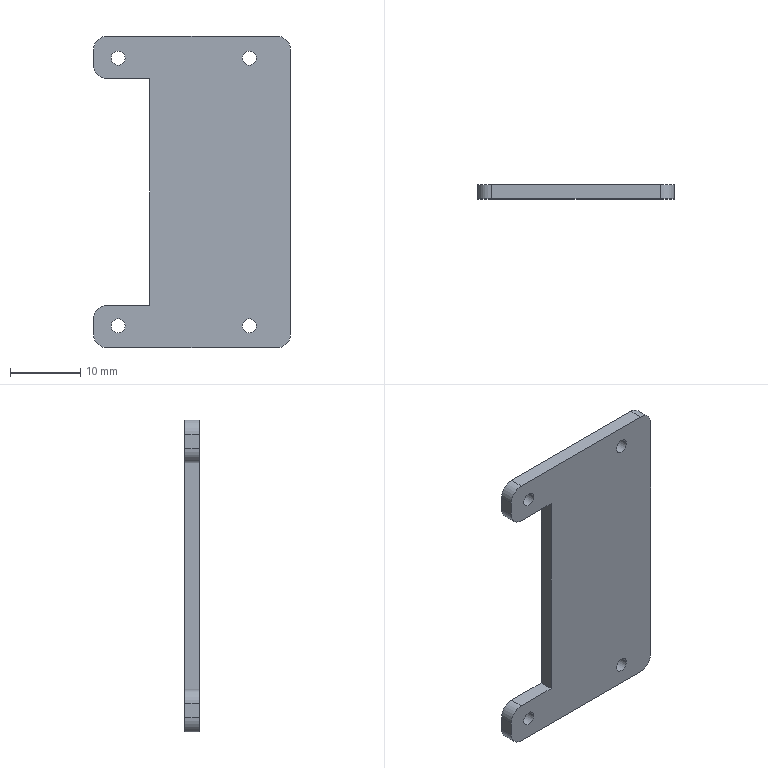Component | SolidWorks | UpperBaffle-1 | 1 solid | 29 faces | box 28.11 x 2 x 44.52 mm | volume 1827 mm3 | plane 15 | cylinder 14 | commonest cylinder face diameters 2 x8 4 x6
build123d program:
from build123d import *

# Parameters (mm, degrees)
BOSS_EXTRUDE1_DEPTH = 2
FILLET1_R           = 2
SKETCH2_R           = 1
CUT_EXTRUDE1_DEPTH  = 10
SKETCH3_W           = 10.322
SKETCH3_H           = 23.58
CUT_EXTRUDE2_DEPTH  = 0.5


with BuildPart() as part:
    # Sketch1 → Boss-Extrude1 (new body)
    with BuildSketch(Plane.XY):
        Polygon((102.385, 21.878), (74.276, 21.878), (74.276, 15.789), (82.305, 15.789), (82.305, -16.558), (74.276, -16.558), (74.276, -22.646), (102.385, -22.646), align=None)
    extrude(amount=BOSS_EXTRUDE1_DEPTH)

    # Fillet1
    fillet1_edges = [part.edges().sort_by_distance(p)[0] for p in [
        (102.385, -22.646, 1),
        (74.276, -22.646, 1),
        (74.276, -16.558, 1),
        (74.276, 15.789, 1),
        (74.276, 21.878, 1),
        (102.385, 21.878, 1),
    ]]
    fillet(fillet1_edges, radius=FILLET1_R)

    # Sketch2 → Cut-Extrude1 (cut)
    with BuildSketch(Plane.XY.offset(2)):
        with Locations((96.517, 18.738)):
            Circle(SKETCH2_R)
        with Locations((77.792, 18.738)):
            Circle(SKETCH2_R)
        with Locations(Location((77.792, -19.506, 0), (0, 0, 180))):
            Circle(SKETCH2_R)
        with Locations(Location((96.517, -19.506, 0), (0, 0, 180))):
            Circle(SKETCH2_R)
    extrude(amount=-CUT_EXTRUDE1_DEPTH, mode=Mode.SUBTRACT)

    # Sketch3 → Cut-Extrude2 (cut)
    with BuildSketch(Plane.XY.offset(2)):
        with Locations((91.241, -0.1111)):
            Rectangle(SKETCH3_W, SKETCH3_H)
    extrude(amount=-CUT_EXTRUDE2_DEPTH, mode=Mode.SUBTRACT)


solid = part.part

# Placed as in the assembly
solid = solid.moved(Location((-18.393, 86.06, 0.5406), (-90, 0, 0)))
STEP:
#1=CARTESIAN_POINT('',(3.115,3.388,0.7893));
#2=VERTEX_POINT('',#1);
#3=CARTESIAN_POINT('',(3.036,3.388,0.7893));
#4=VERTEX_POINT('',#3);
#5=CARTESIAN_POINT('',(3.076,3.388,0.7893));
#6=DIRECTION('',(-0.,-1.,0.));
#7=DIRECTION('',(-1.,0.,0.));
#8=AXIS2_PLACEMENT_3D('',#5,#6,#7);
#9=CIRCLE('',#8,0.03937);
#10=EDGE_CURVE('',#2,#4,#9,.T.);
#11=ORIENTED_EDGE('',*,*,#10,.T.);
#12=CARTESIAN_POINT('',(3.036,3.467,0.7893));
#13=VERTEX_POINT('',#12);
#14=CARTESIAN_POINT('',(3.036,3.073,0.7893));
#15=DIRECTION('',(0.,1.,0.));
#16=VECTOR('',#15,39.37);
#17=LINE('',#14,#16);
#18=EDGE_CURVE('',#4,#13,#17,.T.);
#19=ORIENTED_EDGE('',*,*,#18,.T.);
#20=CARTESIAN_POINT('',(3.115,3.467,0.7893));
#21=VERTEX_POINT('',#20);
#22=CARTESIAN_POINT('',(3.076,3.467,0.7893));
#23=DIRECTION('',(0.,1.,0.));
#24=DIRECTION('',(-1.,0.,0.));
#25=AXIS2_PLACEMENT_3D('',#22,#23,#24);
#26=CIRCLE('',#25,0.03937);
#27=EDGE_CURVE('',#13,#21,#26,.T.);
#28=ORIENTED_EDGE('',*,*,#27,.T.);
#29=CARTESIAN_POINT('',(3.115,3.073,0.7893));
#30=DIRECTION('',(0.,1.,0.));
#31=VECTOR('',#30,39.37);
#32=LINE('',#29,#31);
#33=EDGE_CURVE('',#2,#21,#32,.T.);
#34=ORIENTED_EDGE('',*,*,#33,.F.);
#35=EDGE_LOOP('',(#11,#19,#28,#34));
#36=FACE_OUTER_BOUND('',#35,.T.);
#37=CARTESIAN_POINT('',(3.076,3.073,0.7893));
#38=DIRECTION('',(0.,1.,0.));
#39=DIRECTION('',(1.,0.,0.));
#40=AXIS2_PLACEMENT_3D('',#37,#38,#39);
#41=CYLINDRICAL_SURFACE('',#40,0.03937);
#42=ADVANCED_FACE('',(#36),#41,.F.);
#43=CARTESIAN_POINT('',(2.378,3.388,0.7893));
#44=VERTEX_POINT('',#43);
#45=CARTESIAN_POINT('',(2.299,3.388,0.7893));
#46=VERTEX_POINT('',#45);
#47=CARTESIAN_POINT('',(2.339,3.388,0.7893));
#48=DIRECTION('',(-0.,-1.,0.));
#49=DIRECTION('',(-1.,0.,0.));
#50=AXIS2_PLACEMENT_3D('',#47,#48,#49);
#51=CIRCLE('',#50,0.03937);
#52=EDGE_CURVE('',#44,#46,#51,.T.);
#53=ORIENTED_EDGE('',*,*,#52,.T.);
#54=CARTESIAN_POINT('',(2.299,3.467,0.7893));
#55=VERTEX_POINT('',#54);
#56=CARTESIAN_POINT('',(2.299,3.073,0.7893));
#57=DIRECTION('',(0.,1.,0.));
#58=VECTOR('',#57,39.37);
#59=LINE('',#56,#58);
#60=EDGE_CURVE('',#46,#55,#59,.T.);
#61=ORIENTED_EDGE('',*,*,#60,.T.);
#62=CARTESIAN_POINT('',(2.378,3.467,0.7893));
#63=VERTEX_POINT('',#62);
#64=CARTESIAN_POINT('',(2.339,3.467,0.7893));
#65=DIRECTION('',(0.,1.,0.));
#66=DIRECTION('',(-1.,0.,0.));
#67=AXIS2_PLACEMENT_3D('',#64,#65,#66);
#68=CIRCLE('',#67,0.03937);
#69=EDGE_CURVE('',#55,#63,#68,.T.);
#70=ORIENTED_EDGE('',*,*,#69,.T.);
#71=CARTESIAN_POINT('',(2.378,3.073,0.7893));
#72=DIRECTION('',(0.,1.,0.));
#73=VECTOR('',#72,39.37);
#74=LINE('',#71,#73);
#75=EDGE_CURVE('',#44,#63,#74,.T.);
#76=ORIENTED_EDGE('',*,*,#75,.F.);
#77=EDGE_LOOP('',(#53,#61,#70,#76));
#78=FACE_OUTER_BOUND('',#77,.T.);
#79=CARTESIAN_POINT('',(2.339,3.073,0.7893));
#80=DIRECTION('',(0.,1.,0.));
#81=DIRECTION('',(1.,0.,0.));
#82=AXIS2_PLACEMENT_3D('',#79,#80,#81);
#83=CYLINDRICAL_SURFACE('',#82,0.03937);
#84=ADVANCED_FACE('',(#78),#83,.F.);
#85=CARTESIAN_POINT('',(2.378,3.388,-0.7164));
#86=VERTEX_POINT('',#85);
#87=CARTESIAN_POINT('',(2.299,3.388,-0.7164));
#88=VERTEX_POINT('',#87);
#89=CARTESIAN_POINT('',(2.339,3.388,-0.7164));
#90=DIRECTION('',(-0.,-1.,0.));
#91=DIRECTION('',(-1.,0.,0.));
#92=AXIS2_PLACEMENT_3D('',#89,#90,#91);
#93=CIRCLE('',#92,0.03937);
#94=EDGE_CURVE('',#86,#88,#93,.T.);
#95=ORIENTED_EDGE('',*,*,#94,.T.);
#96=CARTESIAN_POINT('',(2.299,3.467,-0.7164));
#97=VERTEX_POINT('',#96);
#98=CARTESIAN_POINT('',(2.299,3.073,-0.7164));
#99=DIRECTION('',(0.,1.,0.));
#100=VECTOR('',#99,39.37);
#101=LINE('',#98,#100);
#102=EDGE_CURVE('',#88,#97,#101,.T.);
#103=ORIENTED_EDGE('',*,*,#102,.T.);
#104=CARTESIAN_POINT('',(2.378,3.467,-0.7164));
#105=VERTEX_POINT('',#104);
#106=CARTESIAN_POINT('',(2.339,3.467,-0.7164));
#107=DIRECTION('',(0.,1.,0.));
#108=DIRECTION('',(1.,0.,0.));
#109=AXIS2_PLACEMENT_3D('',#106,#107,#108);
#110=CIRCLE('',#109,0.03937);
#111=EDGE_CURVE('',#97,#105,#110,.T.);
#112=ORIENTED_EDGE('',*,*,#111,.T.);
#113=CARTESIAN_POINT('',(2.378,3.073,-0.7164));
#114=DIRECTION('',(0.,1.,0.));
#115=VECTOR('',#114,39.37);
#116=LINE('',#113,#115);
#117=EDGE_CURVE('',#86,#105,#116,.T.);
#118=ORIENTED_EDGE('',*,*,#117,.F.);
#119=EDGE_LOOP('',(#95,#103,#112,#118));
#120=FACE_OUTER_BOUND('',#119,.T.);
#121=CARTESIAN_POINT('',(2.339,3.073,-0.7164));
#122=DIRECTION('',(0.,1.,0.));
#123=DIRECTION('',(1.,0.,0.));
#124=AXIS2_PLACEMENT_3D('',#121,#122,#123);
#125=CYLINDRICAL_SURFACE('',#124,0.03937);
#126=ADVANCED_FACE('',(#120),#125,.F.);
#127=CARTESIAN_POINT('',(3.115,3.388,-0.7164));
#128=VERTEX_POINT('',#127);
#129=CARTESIAN_POINT('',(3.036,3.388,-0.7164));
#130=VERTEX_POINT('',#129);
#131=CARTESIAN_POINT('',(3.076,3.388,-0.7164));
#132=DIRECTION('',(-0.,-1.,0.));
#133=DIRECTION('',(-1.,0.,0.));
#134=AXIS2_PLACEMENT_3D('',#131,#132,#133);
#135=CIRCLE('',#134,0.03937);
#136=EDGE_CURVE('',#128,#130,#135,.T.);
#137=ORIENTED_EDGE('',*,*,#136,.T.);
#138=CARTESIAN_POINT('',(3.036,3.467,-0.7164));
#139=VERTEX_POINT('',#138);
#140=CARTESIAN_POINT('',(3.036,3.073,-0.7164));
#141=DIRECTION('',(0.,1.,0.));
#142=VECTOR('',#141,39.37);
#143=LINE('',#140,#142);
#144=EDGE_CURVE('',#130,#139,#143,.T.);
#145=ORIENTED_EDGE('',*,*,#144,.T.);
#146=CARTESIAN_POINT('',(3.115,3.467,-0.7164));
#147=VERTEX_POINT('',#146);
#148=CARTESIAN_POINT('',(3.076,3.467,-0.7164));
#149=DIRECTION('',(0.,1.,0.));
#150=DIRECTION('',(1.,0.,0.));
#151=AXIS2_PLACEMENT_3D('',#148,#149,#150);
#152=CIRCLE('',#151,0.03937);
#153=EDGE_CURVE('',#139,#147,#152,.T.);
#154=ORIENTED_EDGE('',*,*,#153,.T.);
#155=CARTESIAN_POINT('',(3.115,3.073,-0.7164));
#156=DIRECTION('',(0.,1.,0.));
#157=VECTOR('',#156,39.37);
#158=LINE('',#155,#157);
#159=EDGE_CURVE('',#128,#147,#158,.T.);
#160=ORIENTED_EDGE('',*,*,#159,.F.);
#161=EDGE_LOOP('',(#137,#145,#154,#160));
#162=FACE_OUTER_BOUND('',#161,.T.);
#163=CARTESIAN_POINT('',(3.076,3.073,-0.7164));
#164=DIRECTION('',(0.,1.,0.));
#165=DIRECTION('',(1.,0.,0.));
#166=AXIS2_PLACEMENT_3D('',#163,#164,#165);
#167=CYLINDRICAL_SURFACE('',#166,0.03937);
#168=ADVANCED_FACE('',(#162),#167,.F.);
#169=CARTESIAN_POINT('',(3.307,3.467,0.8341));
#170=VERTEX_POINT('',#169);
#171=CARTESIAN_POINT('',(3.307,3.467,-0.7613));
#172=VERTEX_POINT('',#171);
#173=CARTESIAN_POINT('',(3.307,3.467,-0.84));
#174=DIRECTION('',(0.,0.,-1.));
#175=VECTOR('',#174,39.37);
#176=LINE('',#173,#175);
#177=EDGE_CURVE('',#170,#172,#176,.T.);
#178=ORIENTED_EDGE('',*,*,#177,.F.);
#179=CARTESIAN_POINT('',(3.307,3.388,0.8341));
#180=VERTEX_POINT('',#179);
#181=CARTESIAN_POINT('',(3.307,3.467,0.8341));
#182=DIRECTION('',(-0.,-1.,0.));
#183=VECTOR('',#182,39.37);
#184=LINE('',#181,#183);
#185=EDGE_CURVE('',#170,#180,#184,.T.);
#186=ORIENTED_EDGE('',*,*,#185,.T.);
#187=CARTESIAN_POINT('',(3.307,3.388,-0.7613));
#188=VERTEX_POINT('',#187);
#189=CARTESIAN_POINT('',(3.307,3.388,-0.84));
#190=DIRECTION('',(0.,0.,-1.));
#191=VECTOR('',#190,39.37);
#192=LINE('',#189,#191);
#193=EDGE_CURVE('',#180,#188,#192,.T.);
#194=ORIENTED_EDGE('',*,*,#193,.T.);
#195=CARTESIAN_POINT('',(3.307,3.467,-0.7613));
#196=DIRECTION('',(0.,1.,0.));
#197=VECTOR('',#196,39.37);
#198=LINE('',#195,#197);
#199=EDGE_CURVE('',#188,#172,#198,.T.);
#200=ORIENTED_EDGE('',*,*,#199,.T.);
#201=EDGE_LOOP('',(#178,#186,#194,#200));
#202=FACE_OUTER_BOUND('',#201,.T.);
#203=CARTESIAN_POINT('',(3.307,3.467,-0.84));
#204=DIRECTION('',(-1.,0.,0.));
#205=DIRECTION('',(0.,1.,0.));
#206=AXIS2_PLACEMENT_3D('',#203,#204,#205);
#207=PLANE('',#206);
#208=ADVANCED_FACE('',(#202),#207,.F.);
#209=CARTESIAN_POINT('',(3.228,3.388,-0.84));
#210=VERTEX_POINT('',#209);
#211=CARTESIAN_POINT('',(2.279,3.388,-0.84));
#212=VERTEX_POINT('',#211);
#213=CARTESIAN_POINT('',(3.307,3.388,-0.84));
#214=DIRECTION('',(-1.,0.,-0.));
#215=VECTOR('',#214,39.37);
#216=LINE('',#213,#215);
#217=EDGE_CURVE('',#210,#212,#216,.T.);
#218=ORIENTED_EDGE('',*,*,#217,.T.);
#219=CARTESIAN_POINT('',(2.279,3.467,-0.84));
#220=VERTEX_POINT('',#219);
#221=CARTESIAN_POINT('',(2.279,3.467,-0.84));
#222=DIRECTION('',(0.,1.,0.));
#223=VECTOR('',#222,39.37);
#224=LINE('',#221,#223);
#225=EDGE_CURVE('',#212,#220,#224,.T.);
#226=ORIENTED_EDGE('',*,*,#225,.T.);
#227=CARTESIAN_POINT('',(3.228,3.467,-0.84));
#228=VERTEX_POINT('',#227);
#229=CARTESIAN_POINT('',(3.307,3.467,-0.84));
#230=DIRECTION('',(-1.,0.,-0.));
#231=VECTOR('',#230,39.37);
#232=LINE('',#229,#231);
#233=EDGE_CURVE('',#228,#220,#232,.T.);
#234=ORIENTED_EDGE('',*,*,#233,.F.);
#235=CARTESIAN_POINT('',(3.228,3.467,-0.84));
#236=DIRECTION('',(-0.,-1.,0.));
#237=VECTOR('',#236,39.37);
#238=LINE('',#235,#237);
#239=EDGE_CURVE('',#228,#210,#238,.T.);
#240=ORIENTED_EDGE('',*,*,#239,.T.);
#241=EDGE_LOOP('',(#218,#226,#234,#240));
#242=FACE_OUTER_BOUND('',#241,.T.);
#243=CARTESIAN_POINT('',(3.307,3.467,-0.84));
#244=DIRECTION('',(-0.,0.,1.));
#245=DIRECTION('',(1.,-0.,0.));
#246=AXIS2_PLACEMENT_3D('',#243,#244,#245);
#247=PLANE('',#246);
#248=ADVANCED_FACE('',(#242),#247,.F.);
#249=CARTESIAN_POINT('',(2.2,3.388,-0.7613));
#250=VERTEX_POINT('',#249);
#251=CARTESIAN_POINT('',(2.2,3.388,-0.6791));
#252=VERTEX_POINT('',#251);
#253=CARTESIAN_POINT('',(2.2,3.388,-0.84));
#254=DIRECTION('',(0.,0.,1.));
#255=VECTOR('',#254,39.37);
#256=LINE('',#253,#255);
#257=EDGE_CURVE('',#250,#252,#256,.T.);
#258=ORIENTED_EDGE('',*,*,#257,.T.);
#259=CARTESIAN_POINT('',(2.2,3.467,-0.6791));
#260=VERTEX_POINT('',#259);
#261=CARTESIAN_POINT('',(2.2,3.467,-0.6791));
#262=DIRECTION('',(0.,1.,0.));
#263=VECTOR('',#262,39.37);
#264=LINE('',#261,#263);
#265=EDGE_CURVE('',#252,#260,#264,.T.);
#266=ORIENTED_EDGE('',*,*,#265,.T.);
#267=CARTESIAN_POINT('',(2.2,3.467,-0.7613));
#268=VERTEX_POINT('',#267);
#269=CARTESIAN_POINT('',(2.2,3.467,-0.84));
#270=DIRECTION('',(0.,0.,1.));
#271=VECTOR('',#270,39.37);
#272=LINE('',#269,#271);
#273=EDGE_CURVE('',#268,#260,#272,.T.);
#274=ORIENTED_EDGE('',*,*,#273,.F.);
#275=CARTESIAN_POINT('',(2.2,3.467,-0.7613));
#276=DIRECTION('',(-0.,-1.,0.));
#277=VECTOR('',#276,39.37);
#278=LINE('',#275,#277);
#279=EDGE_CURVE('',#268,#250,#278,.T.);
#280=ORIENTED_EDGE('',*,*,#279,.T.);
#281=EDGE_LOOP('',(#258,#266,#274,#280));
#282=FACE_OUTER_BOUND('',#281,.T.);
#283=CARTESIAN_POINT('',(2.2,3.467,-0.84));
#284=DIRECTION('',(1.,-0.,0.));
#285=DIRECTION('',(-0.,-1.,0.));
#286=AXIS2_PLACEMENT_3D('',#283,#284,#285);
#287=PLANE('',#286);
#288=ADVANCED_FACE('',(#282),#287,.F.);
#289=CARTESIAN_POINT('',(2.279,3.467,-0.6003));
#290=VERTEX_POINT('',#289);
#291=CARTESIAN_POINT('',(2.516,3.467,-0.6003));
#292=VERTEX_POINT('',#291);
#293=CARTESIAN_POINT('',(2.2,3.467,-0.6003));
#294=DIRECTION('',(1.,-0.,0.));
#295=VECTOR('',#294,39.37);
#296=LINE('',#293,#295);
#297=EDGE_CURVE('',#290,#292,#296,.T.);
#298=ORIENTED_EDGE('',*,*,#297,.F.);
#299=CARTESIAN_POINT('',(2.279,3.388,-0.6003));
#300=VERTEX_POINT('',#299);
#301=CARTESIAN_POINT('',(2.279,3.467,-0.6003));
#302=DIRECTION('',(-0.,-1.,0.));
#303=VECTOR('',#302,39.37);
#304=LINE('',#301,#303);
#305=EDGE_CURVE('',#290,#300,#304,.T.);
#306=ORIENTED_EDGE('',*,*,#305,.T.);
#307=CARTESIAN_POINT('',(2.516,3.388,-0.6003));
#308=VERTEX_POINT('',#307);
#309=CARTESIAN_POINT('',(2.2,3.388,-0.6003));
#310=DIRECTION('',(1.,-0.,0.));
#311=VECTOR('',#310,39.37);
#312=LINE('',#309,#311);
#313=EDGE_CURVE('',#300,#308,#312,.T.);
#314=ORIENTED_EDGE('',*,*,#313,.T.);
#315=CARTESIAN_POINT('',(2.516,3.467,-0.6003));
#316=DIRECTION('',(-0.,-1.,0.));
#317=VECTOR('',#316,39.37);
#318=LINE('',#315,#317);
#319=EDGE_CURVE('',#292,#308,#318,.T.);
#320=ORIENTED_EDGE('',*,*,#319,.F.);
#321=EDGE_LOOP('',(#298,#306,#314,#320));
#322=FACE_OUTER_BOUND('',#321,.T.);
#323=CARTESIAN_POINT('',(2.2,3.467,-0.6003));
#324=DIRECTION('',(0.,-0.,-1.));
#325=DIRECTION('',(-1.,0.,-0.));
#326=AXIS2_PLACEMENT_3D('',#323,#324,#325);
#327=PLANE('',#326);
#328=ADVANCED_FACE('',(#322),#327,.F.);
#329=CARTESIAN_POINT('',(2.516,3.388,0.6732));
#330=VERTEX_POINT('',#329);
#331=CARTESIAN_POINT('',(2.516,3.388,-0.6003));
#332=DIRECTION('',(0.,0.,1.));
#333=VECTOR('',#332,39.37);
#334=LINE('',#331,#333);
#335=EDGE_CURVE('',#308,#330,#334,.T.);
#336=ORIENTED_EDGE('',*,*,#335,.T.);
#337=CARTESIAN_POINT('',(2.516,3.467,0.6732));
#338=VERTEX_POINT('',#337);
#339=CARTESIAN_POINT('',(2.516,3.467,0.6732));
#340=DIRECTION('',(-0.,-1.,0.));
#341=VECTOR('',#340,39.37);
#342=LINE('',#339,#341);
#343=EDGE_CURVE('',#338,#330,#342,.T.);
#344=ORIENTED_EDGE('',*,*,#343,.F.);
#345=CARTESIAN_POINT('',(2.516,3.467,-0.6003));
#346=DIRECTION('',(0.,0.,1.));
#347=VECTOR('',#346,39.37);
#348=LINE('',#345,#347);
#349=EDGE_CURVE('',#292,#338,#348,.T.);
#350=ORIENTED_EDGE('',*,*,#349,.F.);
#351=ORIENTED_EDGE('',*,*,#319,.T.);
#352=EDGE_LOOP('',(#336,#344,#350,#351));
#353=FACE_OUTER_BOUND('',#352,.T.);
#354=CARTESIAN_POINT('',(2.516,3.467,-0.6003));
#355=DIRECTION('',(1.,-0.,0.));
#356=DIRECTION('',(-0.,-1.,0.));
#357=AXIS2_PLACEMENT_3D('',#354,#355,#356);
#358=PLANE('',#357);
#359=ADVANCED_FACE('',(#353),#358,.F.);
#360=CARTESIAN_POINT('',(2.279,3.388,0.6732));
#361=VERTEX_POINT('',#360);
#362=CARTESIAN_POINT('',(2.2,3.388,0.6732));
#363=DIRECTION('',(-1.,0.,0.));
#364=VECTOR('',#363,39.37);
#365=LINE('',#362,#364);
#366=EDGE_CURVE('',#330,#361,#365,.T.);
#367=ORIENTED_EDGE('',*,*,#366,.T.);
#368=CARTESIAN_POINT('',(2.279,3.467,0.6732));
#369=VERTEX_POINT('',#368);
#370=CARTESIAN_POINT('',(2.279,3.467,0.6732));
#371=DIRECTION('',(0.,1.,0.));
#372=VECTOR('',#371,39.37);
#373=LINE('',#370,#372);
#374=EDGE_CURVE('',#361,#369,#373,.T.);
#375=ORIENTED_EDGE('',*,*,#374,.T.);
#376=CARTESIAN_POINT('',(2.2,3.467,0.6732));
#377=DIRECTION('',(-1.,0.,0.));
#378=VECTOR('',#377,39.37);
#379=LINE('',#376,#378);
#380=EDGE_CURVE('',#338,#369,#379,.T.);
#381=ORIENTED_EDGE('',*,*,#380,.F.);
#382=ORIENTED_EDGE('',*,*,#343,.T.);
#383=EDGE_LOOP('',(#367,#375,#381,#382));
#384=FACE_OUTER_BOUND('',#383,.T.);
#385=CARTESIAN_POINT('',(2.2,3.467,0.6732));
#386=DIRECTION('',(0.,-0.,1.));
#387=DIRECTION('',(1.,-0.,-0.));
#388=AXIS2_PLACEMENT_3D('',#385,#386,#387);
#389=PLANE('',#388);
#390=ADVANCED_FACE('',(#384),#389,.F.);
#391=CARTESIAN_POINT('',(2.2,3.388,0.7519));
#392=VERTEX_POINT('',#391);
#393=CARTESIAN_POINT('',(2.2,3.388,0.8341));
#394=VERTEX_POINT('',#393);
#395=CARTESIAN_POINT('',(2.2,3.388,0.6732));
#396=DIRECTION('',(-0.,0.,1.));
#397=VECTOR('',#396,39.37);
#398=LINE('',#395,#397);
#399=EDGE_CURVE('',#392,#394,#398,.T.);
#400=ORIENTED_EDGE('',*,*,#399,.T.);
#401=CARTESIAN_POINT('',(2.2,3.467,0.8341));
#402=VERTEX_POINT('',#401);
#403=CARTESIAN_POINT('',(2.2,3.467,0.8341));
#404=DIRECTION('',(0.,1.,0.));
#405=VECTOR('',#404,39.37);
#406=LINE('',#403,#405);
#407=EDGE_CURVE('',#394,#402,#406,.T.);
#408=ORIENTED_EDGE('',*,*,#407,.T.);
#409=CARTESIAN_POINT('',(2.2,3.467,0.7519));
#410=VERTEX_POINT('',#409);
#411=CARTESIAN_POINT('',(2.2,3.467,0.6732));
#412=DIRECTION('',(-0.,0.,1.));
#413=VECTOR('',#412,39.37);
#414=LINE('',#411,#413);
#415=EDGE_CURVE('',#410,#402,#414,.T.);
#416=ORIENTED_EDGE('',*,*,#415,.F.);
#417=CARTESIAN_POINT('',(2.2,3.467,0.7519));
#418=DIRECTION('',(-0.,-1.,0.));
#419=VECTOR('',#418,39.37);
#420=LINE('',#417,#419);
#421=EDGE_CURVE('',#410,#392,#420,.T.);
#422=ORIENTED_EDGE('',*,*,#421,.T.);
#423=EDGE_LOOP('',(#400,#408,#416,#422));
#424=FACE_OUTER_BOUND('',#423,.T.);
#425=CARTESIAN_POINT('',(2.2,3.467,0.6732));
#426=DIRECTION('',(1.,-0.,0.));
#427=DIRECTION('',(0.,-0.,-1.));
#428=AXIS2_PLACEMENT_3D('',#425,#426,#427);
#429=PLANE('',#428);
#430=ADVANCED_FACE('',(#424),#429,.F.);
#431=CARTESIAN_POINT('',(2.279,3.467,0.9129));
#432=VERTEX_POINT('',#431);
#433=CARTESIAN_POINT('',(3.228,3.467,0.9129));
#434=VERTEX_POINT('',#433);
#435=CARTESIAN_POINT('',(3.307,3.467,0.9129));
#436=DIRECTION('',(1.,-0.,-0.));
#437=VECTOR('',#436,39.37);
#438=LINE('',#435,#437);
#439=EDGE_CURVE('',#432,#434,#438,.T.);
#440=ORIENTED_EDGE('',*,*,#439,.F.);
#441=CARTESIAN_POINT('',(2.279,3.388,0.9129));
#442=VERTEX_POINT('',#441);
#443=CARTESIAN_POINT('',(2.279,3.467,0.9129));
#444=DIRECTION('',(-0.,-1.,0.));
#445=VECTOR('',#444,39.37);
#446=LINE('',#443,#445);
#447=EDGE_CURVE('',#432,#442,#446,.T.);
#448=ORIENTED_EDGE('',*,*,#447,.T.);
#449=CARTESIAN_POINT('',(3.228,3.388,0.9129));
#450=VERTEX_POINT('',#449);
#451=CARTESIAN_POINT('',(3.307,3.388,0.9129));
#452=DIRECTION('',(1.,-0.,-0.));
#453=VECTOR('',#452,39.37);
#454=LINE('',#451,#453);
#455=EDGE_CURVE('',#442,#450,#454,.T.);
#456=ORIENTED_EDGE('',*,*,#455,.T.);
#457=CARTESIAN_POINT('',(3.228,3.467,0.9129));
#458=DIRECTION('',(0.,1.,0.));
#459=VECTOR('',#458,39.37);
#460=LINE('',#457,#459);
#461=EDGE_CURVE('',#450,#434,#460,.T.);
#462=ORIENTED_EDGE('',*,*,#461,.T.);
#463=EDGE_LOOP('',(#440,#448,#456,#462));
#464=FACE_OUTER_BOUND('',#463,.T.);
#465=CARTESIAN_POINT('',(3.307,3.467,0.9129));
#466=DIRECTION('',(-0.,0.,-1.));
#467=DIRECTION('',(-1.,0.,0.));
#468=AXIS2_PLACEMENT_3D('',#465,#466,#467);
#469=PLANE('',#468);
#470=ADVANCED_FACE('',(#464),#469,.F.);
#471=CARTESIAN_POINT('',(3.071,3.467,-0.4385));
#472=VERTEX_POINT('',#471);
#473=CARTESIAN_POINT('',(2.665,3.467,-0.4385));
#474=VERTEX_POINT('',#473);
#475=CARTESIAN_POINT('',(3.071,3.467,-0.4385));
#476=DIRECTION('',(-1.,0.,0.));
#477=VECTOR('',#476,39.37);
#478=LINE('',#475,#477);
#479=EDGE_CURVE('',#472,#474,#478,.T.);
#480=ORIENTED_EDGE('',*,*,#479,.F.);
#481=CARTESIAN_POINT('',(3.071,3.467,0.4898));
#482=VERTEX_POINT('',#481);
#483=CARTESIAN_POINT('',(3.071,3.467,-0.4385));
#484=DIRECTION('',(0.,0.,-1.));
#485=VECTOR('',#484,39.37);
#486=LINE('',#483,#485);
#487=EDGE_CURVE('',#482,#472,#486,.T.);
#488=ORIENTED_EDGE('',*,*,#487,.F.);
#489=CARTESIAN_POINT('',(2.665,3.467,0.4898));
#490=VERTEX_POINT('',#489);
#491=CARTESIAN_POINT('',(3.071,3.467,0.4898));
#492=DIRECTION('',(1.,-0.,-0.));
#493=VECTOR('',#492,39.37);
#494=LINE('',#491,#493);
#495=EDGE_CURVE('',#490,#482,#494,.T.);
#496=ORIENTED_EDGE('',*,*,#495,.F.);
#497=CARTESIAN_POINT('',(2.665,3.467,-0.4385));
#498=DIRECTION('',(0.,0.,1.));
#499=VECTOR('',#498,39.37);
#500=LINE('',#497,#499);
#501=EDGE_CURVE('',#474,#490,#500,.T.);
#502=ORIENTED_EDGE('',*,*,#501,.F.);
#503=EDGE_LOOP('',(#480,#488,#496,#502));
#504=FACE_BOUND('',#503,.T.);
#505=CARTESIAN_POINT('',(3.076,3.467,0.7893));
#506=DIRECTION('',(0.,1.,0.));
#507=DIRECTION('',(-1.,0.,0.));
#508=AXIS2_PLACEMENT_3D('',#505,#506,#507);
#509=CIRCLE('',#508,0.03937);
#510=EDGE_CURVE('',#21,#13,#509,.T.);
#511=ORIENTED_EDGE('',*,*,#510,.F.);
#512=ORIENTED_EDGE('',*,*,#27,.F.);
#513=EDGE_LOOP('',(#511,#512));
#514=FACE_BOUND('',#513,.T.);
#515=CARTESIAN_POINT('',(2.339,3.467,0.7893));
#516=DIRECTION('',(0.,1.,0.));
#517=DIRECTION('',(-1.,0.,0.));
#518=AXIS2_PLACEMENT_3D('',#515,#516,#517);
#519=CIRCLE('',#518,0.03937);
#520=EDGE_CURVE('',#63,#55,#519,.T.);
#521=ORIENTED_EDGE('',*,*,#520,.F.);
#522=ORIENTED_EDGE('',*,*,#69,.F.);
#523=EDGE_LOOP('',(#521,#522));
#524=FACE_BOUND('',#523,.T.);
#525=CARTESIAN_POINT('',(2.339,3.467,-0.7164));
#526=DIRECTION('',(0.,1.,0.));
#527=DIRECTION('',(1.,0.,0.));
#528=AXIS2_PLACEMENT_3D('',#525,#526,#527);
#529=CIRCLE('',#528,0.03937);
#530=EDGE_CURVE('',#105,#97,#529,.T.);
#531=ORIENTED_EDGE('',*,*,#530,.F.);
#532=ORIENTED_EDGE('',*,*,#111,.F.);
#533=EDGE_LOOP('',(#531,#532));
#534=FACE_BOUND('',#533,.T.);
#535=CARTESIAN_POINT('',(3.076,3.467,-0.7164));
#536=DIRECTION('',(0.,1.,0.));
#537=DIRECTION('',(1.,0.,0.));
#538=AXIS2_PLACEMENT_3D('',#535,#536,#537);
#539=CIRCLE('',#538,0.03937);
#540=EDGE_CURVE('',#147,#139,#539,.T.);
#541=ORIENTED_EDGE('',*,*,#540,.F.);
#542=ORIENTED_EDGE('',*,*,#153,.F.);
#543=EDGE_LOOP('',(#541,#542));
#544=FACE_BOUND('',#543,.T.);
#545=ORIENTED_EDGE('',*,*,#415,.T.);
#546=CARTESIAN_POINT('',(2.279,3.467,0.8341));
#547=DIRECTION('',(0.,1.,0.));
#548=DIRECTION('',(-1.,0.,0.));
#549=AXIS2_PLACEMENT_3D('',#546,#547,#548);
#550=CIRCLE('',#549,0.07874);
#551=EDGE_CURVE('',#402,#432,#550,.T.);
#552=ORIENTED_EDGE('',*,*,#551,.T.);
#553=ORIENTED_EDGE('',*,*,#439,.T.);
#554=CARTESIAN_POINT('',(3.228,3.467,0.8341));
#555=DIRECTION('',(0.,1.,0.));
#556=DIRECTION('',(-1.,0.,0.));
#557=AXIS2_PLACEMENT_3D('',#554,#555,#556);
#558=CIRCLE('',#557,0.07874);
#559=EDGE_CURVE('',#434,#170,#558,.T.);
#560=ORIENTED_EDGE('',*,*,#559,.T.);
#561=ORIENTED_EDGE('',*,*,#177,.T.);
#562=CARTESIAN_POINT('',(3.228,3.467,-0.7613));
#563=DIRECTION('',(0.,1.,0.));
#564=DIRECTION('',(-1.,0.,0.));
#565=AXIS2_PLACEMENT_3D('',#562,#563,#564);
#566=CIRCLE('',#565,0.07874);
#567=EDGE_CURVE('',#172,#228,#566,.T.);
#568=ORIENTED_EDGE('',*,*,#567,.T.);
#569=ORIENTED_EDGE('',*,*,#233,.T.);
#570=CARTESIAN_POINT('',(2.279,3.467,-0.7613));
#571=DIRECTION('',(0.,1.,0.));
#572=DIRECTION('',(-1.,0.,0.));
#573=AXIS2_PLACEMENT_3D('',#570,#571,#572);
#574=CIRCLE('',#573,0.07874);
#575=EDGE_CURVE('',#220,#268,#574,.T.);
#576=ORIENTED_EDGE('',*,*,#575,.T.);
#577=ORIENTED_EDGE('',*,*,#273,.T.);
#578=CARTESIAN_POINT('',(2.279,3.467,-0.6791));
#579=DIRECTION('',(0.,1.,0.));
#580=DIRECTION('',(-1.,0.,0.));
#581=AXIS2_PLACEMENT_3D('',#578,#579,#580);
#582=CIRCLE('',#581,0.07874);
#583=EDGE_CURVE('',#260,#290,#582,.T.);
#584=ORIENTED_EDGE('',*,*,#583,.T.);
#585=ORIENTED_EDGE('',*,*,#297,.T.);
#586=ORIENTED_EDGE('',*,*,#349,.T.);
#587=ORIENTED_EDGE('',*,*,#380,.T.);
#588=CARTESIAN_POINT('',(2.279,3.467,0.7519));
#589=DIRECTION('',(0.,1.,0.));
#590=DIRECTION('',(-1.,0.,0.));
#591=AXIS2_PLACEMENT_3D('',#588,#589,#590);
#592=CIRCLE('',#591,0.07874);
#593=EDGE_CURVE('',#369,#410,#592,.T.);
#594=ORIENTED_EDGE('',*,*,#593,.T.);
#595=EDGE_LOOP('',(#545,#552,#553,#560,#561,#568,#569,#576,#577,#584,#585,#586,#587,#594));
#596=FACE_OUTER_BOUND('',#595,.T.);
#597=CARTESIAN_POINT('',(-0.7241,3.467,0.02128));
#598=DIRECTION('',(-0.,-1.,0.));
#599=DIRECTION('',(-1.,0.,0.));
#600=AXIS2_PLACEMENT_3D('',#597,#598,#599);
#601=PLANE('',#600);
#602=ADVANCED_FACE('',(#504,#514,#524,#534,#544,#596),#601,.F.);
#603=ORIENTED_EDGE('',*,*,#10,.F.);
#604=CARTESIAN_POINT('',(3.076,3.388,0.7893));
#605=DIRECTION('',(-0.,-1.,0.));
#606=DIRECTION('',(-1.,0.,0.));
#607=AXIS2_PLACEMENT_3D('',#604,#605,#606);
#608=CIRCLE('',#607,0.03937);
#609=EDGE_CURVE('',#4,#2,#608,.T.);
#610=ORIENTED_EDGE('',*,*,#609,.F.);
#611=EDGE_LOOP('',(#603,#610));
#612=FACE_BOUND('',#611,.T.);
#613=ORIENTED_EDGE('',*,*,#52,.F.);
#614=CARTESIAN_POINT('',(2.339,3.388,0.7893));
#615=DIRECTION('',(-0.,-1.,0.));
#616=DIRECTION('',(-1.,0.,0.));
#617=AXIS2_PLACEMENT_3D('',#614,#615,#616);
#618=CIRCLE('',#617,0.03937);
#619=EDGE_CURVE('',#46,#44,#618,.T.);
#620=ORIENTED_EDGE('',*,*,#619,.F.);
#621=EDGE_LOOP('',(#613,#620));
#622=FACE_BOUND('',#621,.T.);
#623=ORIENTED_EDGE('',*,*,#94,.F.);
#624=CARTESIAN_POINT('',(2.339,3.388,-0.7164));
#625=DIRECTION('',(-0.,-1.,0.));
#626=DIRECTION('',(-1.,0.,0.));
#627=AXIS2_PLACEMENT_3D('',#624,#625,#626);
#628=CIRCLE('',#627,0.03937);
#629=EDGE_CURVE('',#88,#86,#628,.T.);
#630=ORIENTED_EDGE('',*,*,#629,.F.);
#631=EDGE_LOOP('',(#623,#630));
#632=FACE_BOUND('',#631,.T.);
#633=ORIENTED_EDGE('',*,*,#136,.F.);
#634=CARTESIAN_POINT('',(3.076,3.388,-0.7164));
#635=DIRECTION('',(-0.,-1.,0.));
#636=DIRECTION('',(-1.,0.,0.));
#637=AXIS2_PLACEMENT_3D('',#634,#635,#636);
#638=CIRCLE('',#637,0.03937);
#639=EDGE_CURVE('',#130,#128,#638,.T.);
#640=ORIENTED_EDGE('',*,*,#639,.F.);
#641=EDGE_LOOP('',(#633,#640));
#642=FACE_BOUND('',#641,.T.);
#643=ORIENTED_EDGE('',*,*,#455,.F.);
#644=CARTESIAN_POINT('',(2.279,3.388,0.8341));
#645=DIRECTION('',(-0.,-1.,0.));
#646=DIRECTION('',(-1.,0.,0.));
#647=AXIS2_PLACEMENT_3D('',#644,#645,#646);
#648=CIRCLE('',#647,0.07874);
#649=EDGE_CURVE('',#442,#394,#648,.T.);
#650=ORIENTED_EDGE('',*,*,#649,.T.);
#651=ORIENTED_EDGE('',*,*,#399,.F.);
#652=CARTESIAN_POINT('',(2.279,3.388,0.7519));
#653=DIRECTION('',(-0.,-1.,0.));
#654=DIRECTION('',(-1.,0.,0.));
#655=AXIS2_PLACEMENT_3D('',#652,#653,#654);
#656=CIRCLE('',#655,0.07874);
#657=EDGE_CURVE('',#392,#361,#656,.T.);
#658=ORIENTED_EDGE('',*,*,#657,.T.);
#659=ORIENTED_EDGE('',*,*,#366,.F.);
#660=ORIENTED_EDGE('',*,*,#335,.F.);
#661=ORIENTED_EDGE('',*,*,#313,.F.);
#662=CARTESIAN_POINT('',(2.279,3.388,-0.6791));
#663=DIRECTION('',(-0.,-1.,0.));
#664=DIRECTION('',(-1.,0.,0.));
#665=AXIS2_PLACEMENT_3D('',#662,#663,#664);
#666=CIRCLE('',#665,0.07874);
#667=EDGE_CURVE('',#300,#252,#666,.T.);
#668=ORIENTED_EDGE('',*,*,#667,.T.);
#669=ORIENTED_EDGE('',*,*,#257,.F.);
#670=CARTESIAN_POINT('',(2.279,3.388,-0.7613));
#671=DIRECTION('',(-0.,-1.,0.));
#672=DIRECTION('',(-1.,0.,0.));
#673=AXIS2_PLACEMENT_3D('',#670,#671,#672);
#674=CIRCLE('',#673,0.07874);
#675=EDGE_CURVE('',#250,#212,#674,.T.);
#676=ORIENTED_EDGE('',*,*,#675,.T.);
#677=ORIENTED_EDGE('',*,*,#217,.F.);
#678=CARTESIAN_POINT('',(3.228,3.388,-0.7613));
#679=DIRECTION('',(-0.,-1.,0.));
#680=DIRECTION('',(-1.,0.,0.));
#681=AXIS2_PLACEMENT_3D('',#678,#679,#680);
#682=CIRCLE('',#681,0.07874);
#683=EDGE_CURVE('',#210,#188,#682,.T.);
#684=ORIENTED_EDGE('',*,*,#683,.T.);
#685=ORIENTED_EDGE('',*,*,#193,.F.);
#686=CARTESIAN_POINT('',(3.228,3.388,0.8341));
#687=DIRECTION('',(-0.,-1.,0.));
#688=DIRECTION('',(-1.,0.,0.));
#689=AXIS2_PLACEMENT_3D('',#686,#687,#688);
#690=CIRCLE('',#689,0.07874);
#691=EDGE_CURVE('',#180,#450,#690,.T.);
#692=ORIENTED_EDGE('',*,*,#691,.T.);
#693=EDGE_LOOP('',(#643,#650,#651,#658,#659,#660,#661,#668,#669,#676,#677,#684,#685,#692));
#694=FACE_OUTER_BOUND('',#693,.T.);
#695=CARTESIAN_POINT('',(-0.7241,3.388,0.02128));
#696=DIRECTION('',(-0.,-1.,0.));
#697=DIRECTION('',(-1.,0.,0.));
#698=AXIS2_PLACEMENT_3D('',#695,#696,#697);
#699=PLANE('',#698);
#700=ADVANCED_FACE('',(#612,#622,#632,#642,#694),#699,.T.);
#701=ORIENTED_EDGE('',*,*,#551,.F.);
#702=ORIENTED_EDGE('',*,*,#407,.F.);
#703=ORIENTED_EDGE('',*,*,#649,.F.);
#704=ORIENTED_EDGE('',*,*,#447,.F.);
#705=EDGE_LOOP('',(#701,#702,#703,#704));
#706=FACE_OUTER_BOUND('',#705,.T.);
#707=CARTESIAN_POINT('',(2.279,3.467,0.8341));
#708=DIRECTION('',(-0.,-1.,0.));
#709=DIRECTION('',(-1.,0.,0.));
#710=AXIS2_PLACEMENT_3D('',#707,#708,#709);
#711=CYLINDRICAL_SURFACE('',#710,0.07874);
#712=ADVANCED_FACE('',(#706),#711,.T.);
#713=ORIENTED_EDGE('',*,*,#593,.F.);
#714=ORIENTED_EDGE('',*,*,#374,.F.);
#715=ORIENTED_EDGE('',*,*,#657,.F.);
#716=ORIENTED_EDGE('',*,*,#421,.F.);
#717=EDGE_LOOP('',(#713,#714,#715,#716));
#718=FACE_OUTER_BOUND('',#717,.T.);
#719=CARTESIAN_POINT('',(2.279,3.467,0.7519));
#720=DIRECTION('',(-0.,-1.,0.));
#721=DIRECTION('',(-1.,0.,0.));
#722=AXIS2_PLACEMENT_3D('',#719,#720,#721);
#723=CYLINDRICAL_SURFACE('',#722,0.07874);
#724=ADVANCED_FACE('',(#718),#723,.T.);
#725=ORIENTED_EDGE('',*,*,#583,.F.);
#726=ORIENTED_EDGE('',*,*,#265,.F.);
#727=ORIENTED_EDGE('',*,*,#667,.F.);
#728=ORIENTED_EDGE('',*,*,#305,.F.);
#729=EDGE_LOOP('',(#725,#726,#727,#728));
#730=FACE_OUTER_BOUND('',#729,.T.);
#731=CARTESIAN_POINT('',(2.279,3.467,-0.6791));
#732=DIRECTION('',(-0.,-1.,0.));
#733=DIRECTION('',(-1.,0.,0.));
#734=AXIS2_PLACEMENT_3D('',#731,#732,#733);
#735=CYLINDRICAL_SURFACE('',#734,0.07874);
#736=ADVANCED_FACE('',(#730),#735,.T.);
#737=ORIENTED_EDGE('',*,*,#575,.F.);
#738=ORIENTED_EDGE('',*,*,#225,.F.);
#739=ORIENTED_EDGE('',*,*,#675,.F.);
#740=ORIENTED_EDGE('',*,*,#279,.F.);
#741=EDGE_LOOP('',(#737,#738,#739,#740));
#742=FACE_OUTER_BOUND('',#741,.T.);
#743=CARTESIAN_POINT('',(2.279,3.467,-0.7613));
#744=DIRECTION('',(-0.,-1.,0.));
#745=DIRECTION('',(-1.,0.,0.));
#746=AXIS2_PLACEMENT_3D('',#743,#744,#745);
#747=CYLINDRICAL_SURFACE('',#746,0.07874);
#748=ADVANCED_FACE('',(#742),#747,.T.);
#749=ORIENTED_EDGE('',*,*,#559,.F.);
#750=ORIENTED_EDGE('',*,*,#461,.F.);
#751=ORIENTED_EDGE('',*,*,#691,.F.);
#752=ORIENTED_EDGE('',*,*,#185,.F.);
#753=EDGE_LOOP('',(#749,#750,#751,#752));
#754=FACE_OUTER_BOUND('',#753,.T.);
#755=CARTESIAN_POINT('',(3.228,3.467,0.8341));
#756=DIRECTION('',(-0.,-1.,0.));
#757=DIRECTION('',(-1.,0.,0.));
#758=AXIS2_PLACEMENT_3D('',#755,#756,#757);
#759=CYLINDRICAL_SURFACE('',#758,0.07874);
#760=ADVANCED_FACE('',(#754),#759,.T.);
#761=ORIENTED_EDGE('',*,*,#567,.F.);
#762=ORIENTED_EDGE('',*,*,#199,.F.);
#763=ORIENTED_EDGE('',*,*,#683,.F.);
#764=ORIENTED_EDGE('',*,*,#239,.F.);
#765=EDGE_LOOP('',(#761,#762,#763,#764));
#766=FACE_OUTER_BOUND('',#765,.T.);
#767=CARTESIAN_POINT('',(3.228,3.467,-0.7613));
#768=DIRECTION('',(-0.,-1.,0.));
#769=DIRECTION('',(-1.,0.,0.));
#770=AXIS2_PLACEMENT_3D('',#767,#768,#769);
#771=CYLINDRICAL_SURFACE('',#770,0.07874);
#772=ADVANCED_FACE('',(#766),#771,.T.);
#773=ORIENTED_EDGE('',*,*,#144,.F.);
#774=ORIENTED_EDGE('',*,*,#639,.T.);
#775=ORIENTED_EDGE('',*,*,#159,.T.);
#776=ORIENTED_EDGE('',*,*,#540,.T.);
#777=EDGE_LOOP('',(#773,#774,#775,#776));
#778=FACE_OUTER_BOUND('',#777,.T.);
#779=CARTESIAN_POINT('',(3.076,3.073,-0.7164));
#780=DIRECTION('',(0.,1.,0.));
#781=DIRECTION('',(1.,0.,0.));
#782=AXIS2_PLACEMENT_3D('',#779,#780,#781);
#783=CYLINDRICAL_SURFACE('',#782,0.03937);
#784=ADVANCED_FACE('',(#778),#783,.F.);
#785=ORIENTED_EDGE('',*,*,#102,.F.);
#786=ORIENTED_EDGE('',*,*,#629,.T.);
#787=ORIENTED_EDGE('',*,*,#117,.T.);
#788=ORIENTED_EDGE('',*,*,#530,.T.);
#789=EDGE_LOOP('',(#785,#786,#787,#788));
#790=FACE_OUTER_BOUND('',#789,.T.);
#791=CARTESIAN_POINT('',(2.339,3.073,-0.7164));
#792=DIRECTION('',(0.,1.,0.));
#793=DIRECTION('',(1.,0.,0.));
#794=AXIS2_PLACEMENT_3D('',#791,#792,#793);
#795=CYLINDRICAL_SURFACE('',#794,0.03937);
#796=ADVANCED_FACE('',(#790),#795,.F.);
#797=ORIENTED_EDGE('',*,*,#60,.F.);
#798=ORIENTED_EDGE('',*,*,#619,.T.);
#799=ORIENTED_EDGE('',*,*,#75,.T.);
#800=ORIENTED_EDGE('',*,*,#520,.T.);
#801=EDGE_LOOP('',(#797,#798,#799,#800));
#802=FACE_OUTER_BOUND('',#801,.T.);
#803=CARTESIAN_POINT('',(2.339,3.073,0.7893));
#804=DIRECTION('',(0.,1.,0.));
#805=DIRECTION('',(1.,0.,0.));
#806=AXIS2_PLACEMENT_3D('',#803,#804,#805);
#807=CYLINDRICAL_SURFACE('',#806,0.03937);
#808=ADVANCED_FACE('',(#802),#807,.F.);
#809=ORIENTED_EDGE('',*,*,#18,.F.);
#810=ORIENTED_EDGE('',*,*,#609,.T.);
#811=ORIENTED_EDGE('',*,*,#33,.T.);
#812=ORIENTED_EDGE('',*,*,#510,.T.);
#813=EDGE_LOOP('',(#809,#810,#811,#812));
#814=FACE_OUTER_BOUND('',#813,.T.);
#815=CARTESIAN_POINT('',(3.076,3.073,0.7893));
#816=DIRECTION('',(0.,1.,0.));
#817=DIRECTION('',(1.,0.,0.));
#818=AXIS2_PLACEMENT_3D('',#815,#816,#817);
#819=CYLINDRICAL_SURFACE('',#818,0.03937);
#820=ADVANCED_FACE('',(#814),#819,.F.);
#821=ORIENTED_EDGE('',*,*,#487,.T.);
#822=CARTESIAN_POINT('',(3.071,3.447,-0.4385));
#823=VERTEX_POINT('',#822);
#824=CARTESIAN_POINT('',(3.071,3.447,-0.4385));
#825=DIRECTION('',(0.,1.,0.));
#826=VECTOR('',#825,39.37);
#827=LINE('',#824,#826);
#828=EDGE_CURVE('',#823,#472,#827,.T.);
#829=ORIENTED_EDGE('',*,*,#828,.F.);
#830=CARTESIAN_POINT('',(3.071,3.447,0.4898));
#831=VERTEX_POINT('',#830);
#832=CARTESIAN_POINT('',(3.071,3.447,-0.4385));
#833=DIRECTION('',(0.,0.,-1.));
#834=VECTOR('',#833,39.37);
#835=LINE('',#832,#834);
#836=EDGE_CURVE('',#831,#823,#835,.T.);
#837=ORIENTED_EDGE('',*,*,#836,.F.);
#838=CARTESIAN_POINT('',(3.071,3.447,0.4898));
#839=DIRECTION('',(0.,1.,0.));
#840=VECTOR('',#839,39.37);
#841=LINE('',#838,#840);
#842=EDGE_CURVE('',#831,#482,#841,.T.);
#843=ORIENTED_EDGE('',*,*,#842,.T.);
#844=EDGE_LOOP('',(#821,#829,#837,#843));
#845=FACE_OUTER_BOUND('',#844,.T.);
#846=CARTESIAN_POINT('',(3.071,3.447,-0.4385));
#847=DIRECTION('',(1.,-0.,0.));
#848=DIRECTION('',(-0.,-1.,0.));
#849=AXIS2_PLACEMENT_3D('',#846,#847,#848);
#850=PLANE('',#849);
#851=ADVANCED_FACE('',(#845),#850,.F.);
#852=ORIENTED_EDGE('',*,*,#495,.T.);
#853=ORIENTED_EDGE('',*,*,#842,.F.);
#854=CARTESIAN_POINT('',(2.665,3.447,0.4898));
#855=VERTEX_POINT('',#854);
#856=CARTESIAN_POINT('',(3.071,3.447,0.4898));
#857=DIRECTION('',(1.,-0.,-0.));
#858=VECTOR('',#857,39.37);
#859=LINE('',#856,#858);
#860=EDGE_CURVE('',#855,#831,#859,.T.);
#861=ORIENTED_EDGE('',*,*,#860,.F.);
#862=CARTESIAN_POINT('',(2.665,3.447,0.4898));
#863=DIRECTION('',(0.,1.,0.));
#864=VECTOR('',#863,39.37);
#865=LINE('',#862,#864);
#866=EDGE_CURVE('',#855,#490,#865,.T.);
#867=ORIENTED_EDGE('',*,*,#866,.T.);
#868=EDGE_LOOP('',(#852,#853,#861,#867));
#869=FACE_OUTER_BOUND('',#868,.T.);
#870=CARTESIAN_POINT('',(3.071,3.447,0.4898));
#871=DIRECTION('',(0.,-0.,1.));
#872=DIRECTION('',(1.,-0.,-0.));
#873=AXIS2_PLACEMENT_3D('',#870,#871,#872);
#874=PLANE('',#873);
#875=ADVANCED_FACE('',(#869),#874,.F.);
#876=ORIENTED_EDGE('',*,*,#501,.T.);
#877=ORIENTED_EDGE('',*,*,#866,.F.);
#878=CARTESIAN_POINT('',(2.665,3.447,-0.4385));
#879=VERTEX_POINT('',#878);
#880=CARTESIAN_POINT('',(2.665,3.447,-0.4385));
#881=DIRECTION('',(0.,0.,1.));
#882=VECTOR('',#881,39.37);
#883=LINE('',#880,#882);
#884=EDGE_CURVE('',#879,#855,#883,.T.);
#885=ORIENTED_EDGE('',*,*,#884,.F.);
#886=CARTESIAN_POINT('',(2.665,3.447,-0.4385));
#887=DIRECTION('',(0.,1.,0.));
#888=VECTOR('',#887,39.37);
#889=LINE('',#886,#888);
#890=EDGE_CURVE('',#879,#474,#889,.T.);
#891=ORIENTED_EDGE('',*,*,#890,.T.);
#892=EDGE_LOOP('',(#876,#877,#885,#891));
#893=FACE_OUTER_BOUND('',#892,.T.);
#894=CARTESIAN_POINT('',(2.665,3.447,-0.4385));
#895=DIRECTION('',(-1.,0.,0.));
#896=DIRECTION('',(0.,1.,0.));
#897=AXIS2_PLACEMENT_3D('',#894,#895,#896);
#898=PLANE('',#897);
#899=ADVANCED_FACE('',(#893),#898,.F.);
#900=ORIENTED_EDGE('',*,*,#479,.T.);
#901=ORIENTED_EDGE('',*,*,#890,.F.);
#902=CARTESIAN_POINT('',(3.071,3.447,-0.4385));
#903=DIRECTION('',(-1.,0.,0.));
#904=VECTOR('',#903,39.37);
#905=LINE('',#902,#904);
#906=EDGE_CURVE('',#823,#879,#905,.T.);
#907=ORIENTED_EDGE('',*,*,#906,.F.);
#908=ORIENTED_EDGE('',*,*,#828,.T.);
#909=EDGE_LOOP('',(#900,#901,#907,#908));
#910=FACE_OUTER_BOUND('',#909,.T.);
#911=CARTESIAN_POINT('',(3.071,3.447,-0.4385));
#912=DIRECTION('',(-0.,0.,-1.));
#913=DIRECTION('',(-1.,0.,0.));
#914=AXIS2_PLACEMENT_3D('',#911,#912,#913);
#915=PLANE('',#914);
#916=ADVANCED_FACE('',(#910),#915,.F.);
#917=ORIENTED_EDGE('',*,*,#836,.T.);
#918=ORIENTED_EDGE('',*,*,#906,.T.);
#919=ORIENTED_EDGE('',*,*,#884,.T.);
#920=ORIENTED_EDGE('',*,*,#860,.T.);
#921=EDGE_LOOP('',(#917,#918,#919,#920));
#922=FACE_OUTER_BOUND('',#921,.T.);
#923=CARTESIAN_POINT('',(-0.7241,3.447,0.02128));
#924=DIRECTION('',(-0.,-1.,0.));
#925=DIRECTION('',(-1.,0.,0.));
#926=AXIS2_PLACEMENT_3D('',#923,#924,#925);
#927=PLANE('',#926);
#928=ADVANCED_FACE('',(#922),#927,.F.);
#929=CLOSED_SHELL('',(#42,#84,#126,#168,#208,#248,#288,#328,#359,#390,#430,#470,#602,#700,#712,#724,#736,#748,#760,#772,#784,#796,#808,#820,#851,#875,#899,#916,#928));
#930=MANIFOLD_SOLID_BREP('',#929);
#931=CARTESIAN_POINT('',(0.,0.,0.));
#932=DIRECTION('',(0.,0.,1.));
#933=DIRECTION('',(1.,0.,0.));
#934=AXIS2_PLACEMENT_3D('',#931,#932,#933);
#935=(LENGTH_UNIT()NAMED_UNIT(*)SI_UNIT($,.METRE.));
#936=LENGTH_MEASURE_WITH_UNIT(LENGTH_MEASURE(0.0254),#935);
#937=DIMENSIONAL_EXPONENTS(1.,0.,0.,0.,0.,0.,0.);
#938=(CONVERSION_BASED_UNIT('',#936)LENGTH_UNIT()NAMED_UNIT(#937));
#939=UNCERTAINTY_MEASURE_WITH_UNIT(LENGTH_MEASURE(0.00001),#938,'','');
#940=(NAMED_UNIT(*)PLANE_ANGLE_UNIT()SI_UNIT($,.RADIAN.));
#941=(NAMED_UNIT(*)SI_UNIT($,.STERADIAN.)SOLID_ANGLE_UNIT());
#942=(GEOMETRIC_REPRESENTATION_CONTEXT(3)GLOBAL_UNCERTAINTY_ASSIGNED_CONTEXT((#939))GLOBAL_UNIT_ASSIGNED_CONTEXT((#938,#940,#941))REPRESENTATION_CONTEXT('',''));
#943=ADVANCED_BREP_SHAPE_REPRESENTATION('',(#930,#934),#942);
#944=COLOUR_RGB('',0.7922,0.8196,0.9333);
#945=FILL_AREA_STYLE_COLOUR('',#944);
#946=FILL_AREA_STYLE('',(#945));
#947=SURFACE_STYLE_FILL_AREA(#946);
#948=SURFACE_SIDE_STYLE('',(#947));
#949=SURFACE_STYLE_USAGE(.BOTH.,#948);
#950=PRESENTATION_STYLE_ASSIGNMENT((#949));
#951=STYLED_ITEM('',(#950),#930);
#952=PRESENTATION_LAYER_ASSIGNMENT('','',(#951));
#953=(LENGTH_UNIT()NAMED_UNIT(*)SI_UNIT($,.METRE.));
#954=LENGTH_MEASURE_WITH_UNIT(LENGTH_MEASURE(0.0254),#953);
#955=DIMENSIONAL_EXPONENTS(1.,0.,0.,0.,0.,0.,0.);
#956=(CONVERSION_BASED_UNIT('',#954)LENGTH_UNIT()NAMED_UNIT(#955));
#957=UNCERTAINTY_MEASURE_WITH_UNIT(LENGTH_MEASURE(0.00001),#956,'','');
#958=(NAMED_UNIT(*)PLANE_ANGLE_UNIT()SI_UNIT($,.RADIAN.));
#959=(NAMED_UNIT(*)SI_UNIT($,.STERADIAN.)SOLID_ANGLE_UNIT());
#960=(GEOMETRIC_REPRESENTATION_CONTEXT(3)GLOBAL_UNCERTAINTY_ASSIGNED_CONTEXT((#957))GLOBAL_UNIT_ASSIGNED_CONTEXT((#956,#958,#959))REPRESENTATION_CONTEXT('',''));
#961=MECHANICAL_DESIGN_GEOMETRIC_PRESENTATION_REPRESENTATION('',(#951),#960);